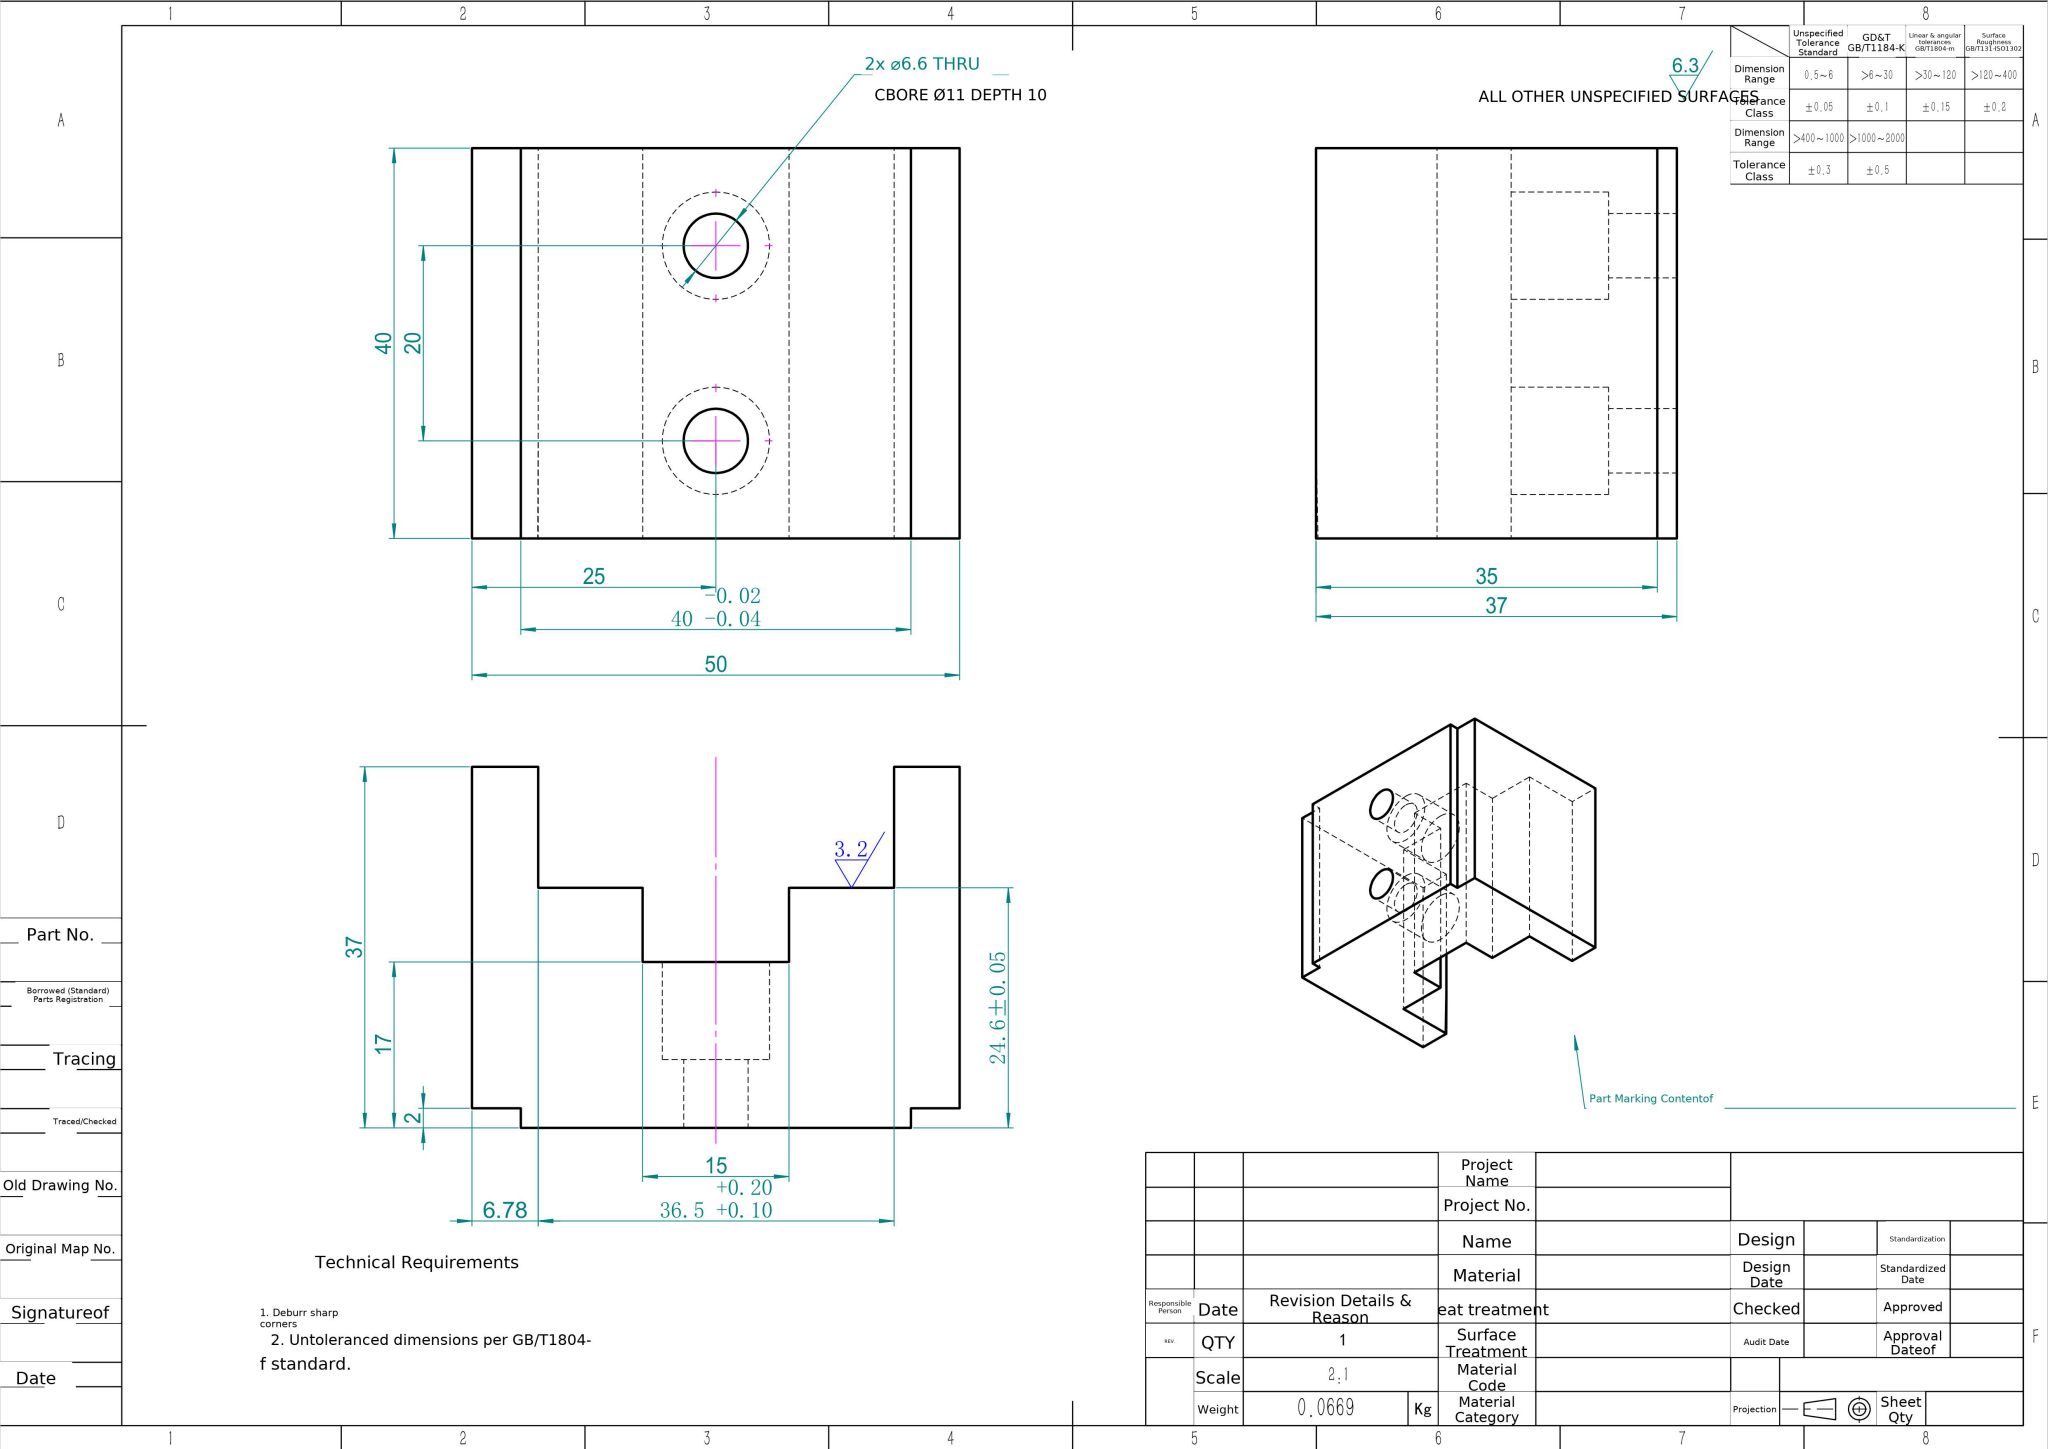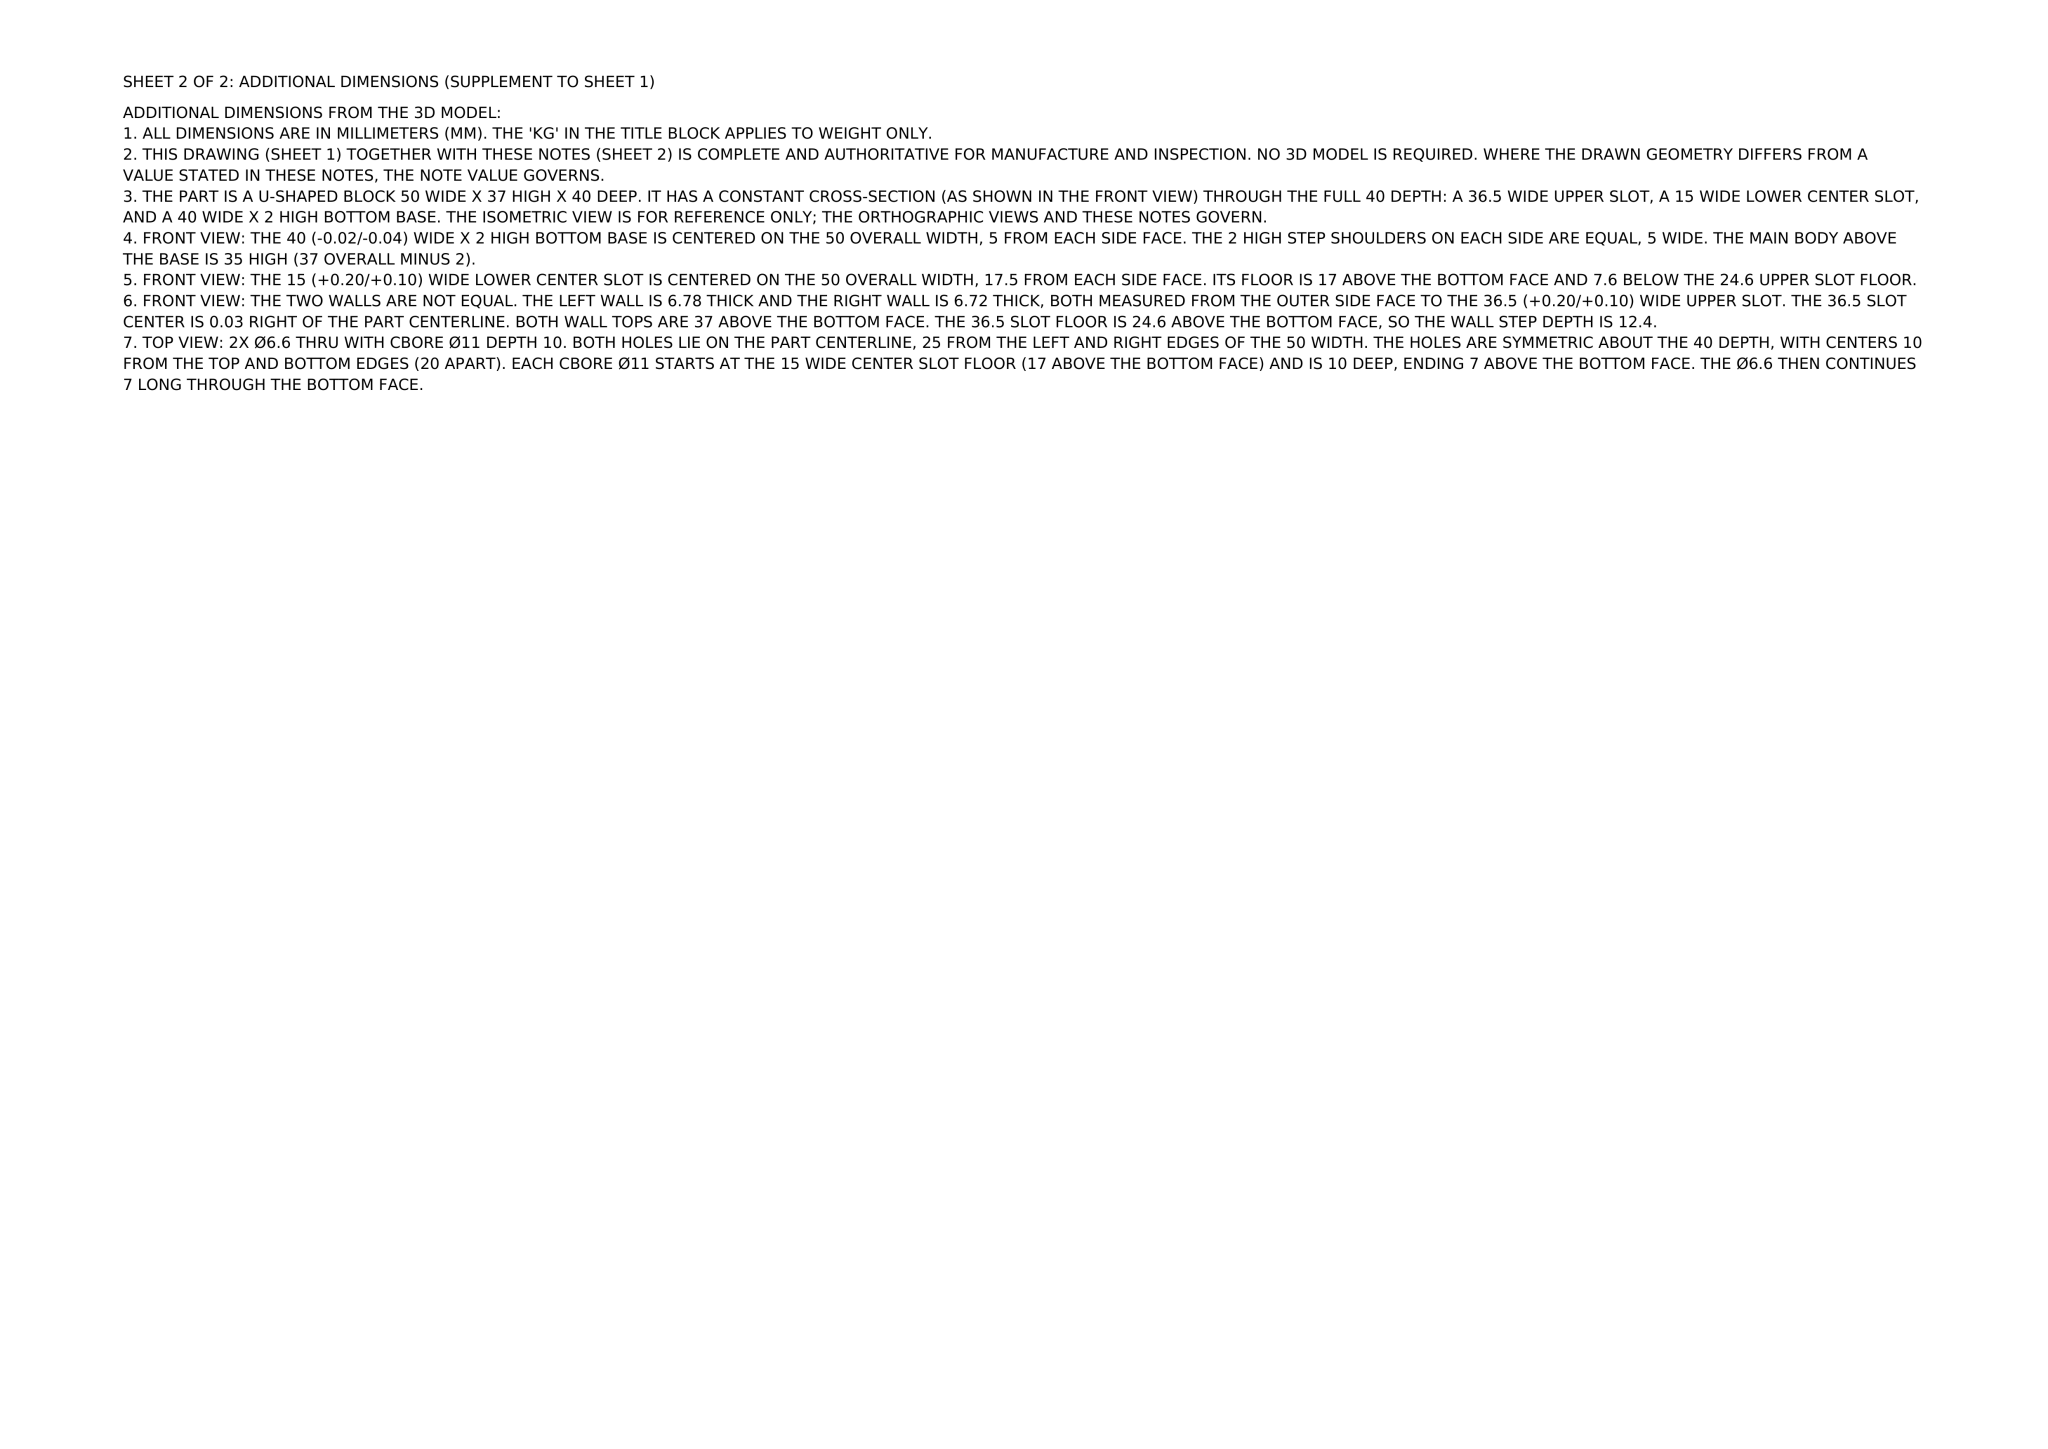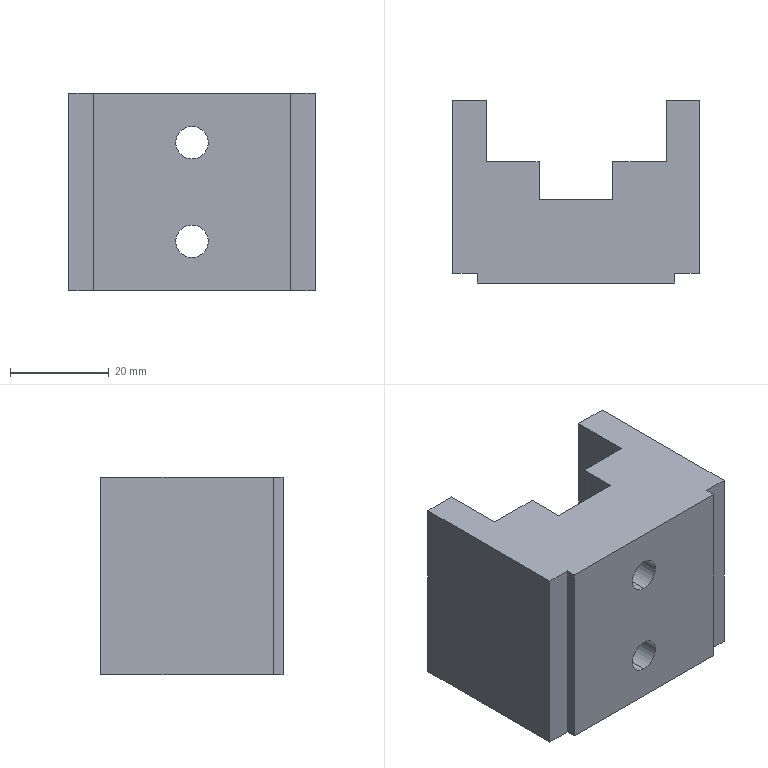Part | NX | mm | 1 solid | 29 faces | box 50 x 37 x 40 mm | volume 48156 mm3 | plane 20 | cylinder 8 | cone 1 | commonest cylinder face diameters 11 x4 6.6 x4